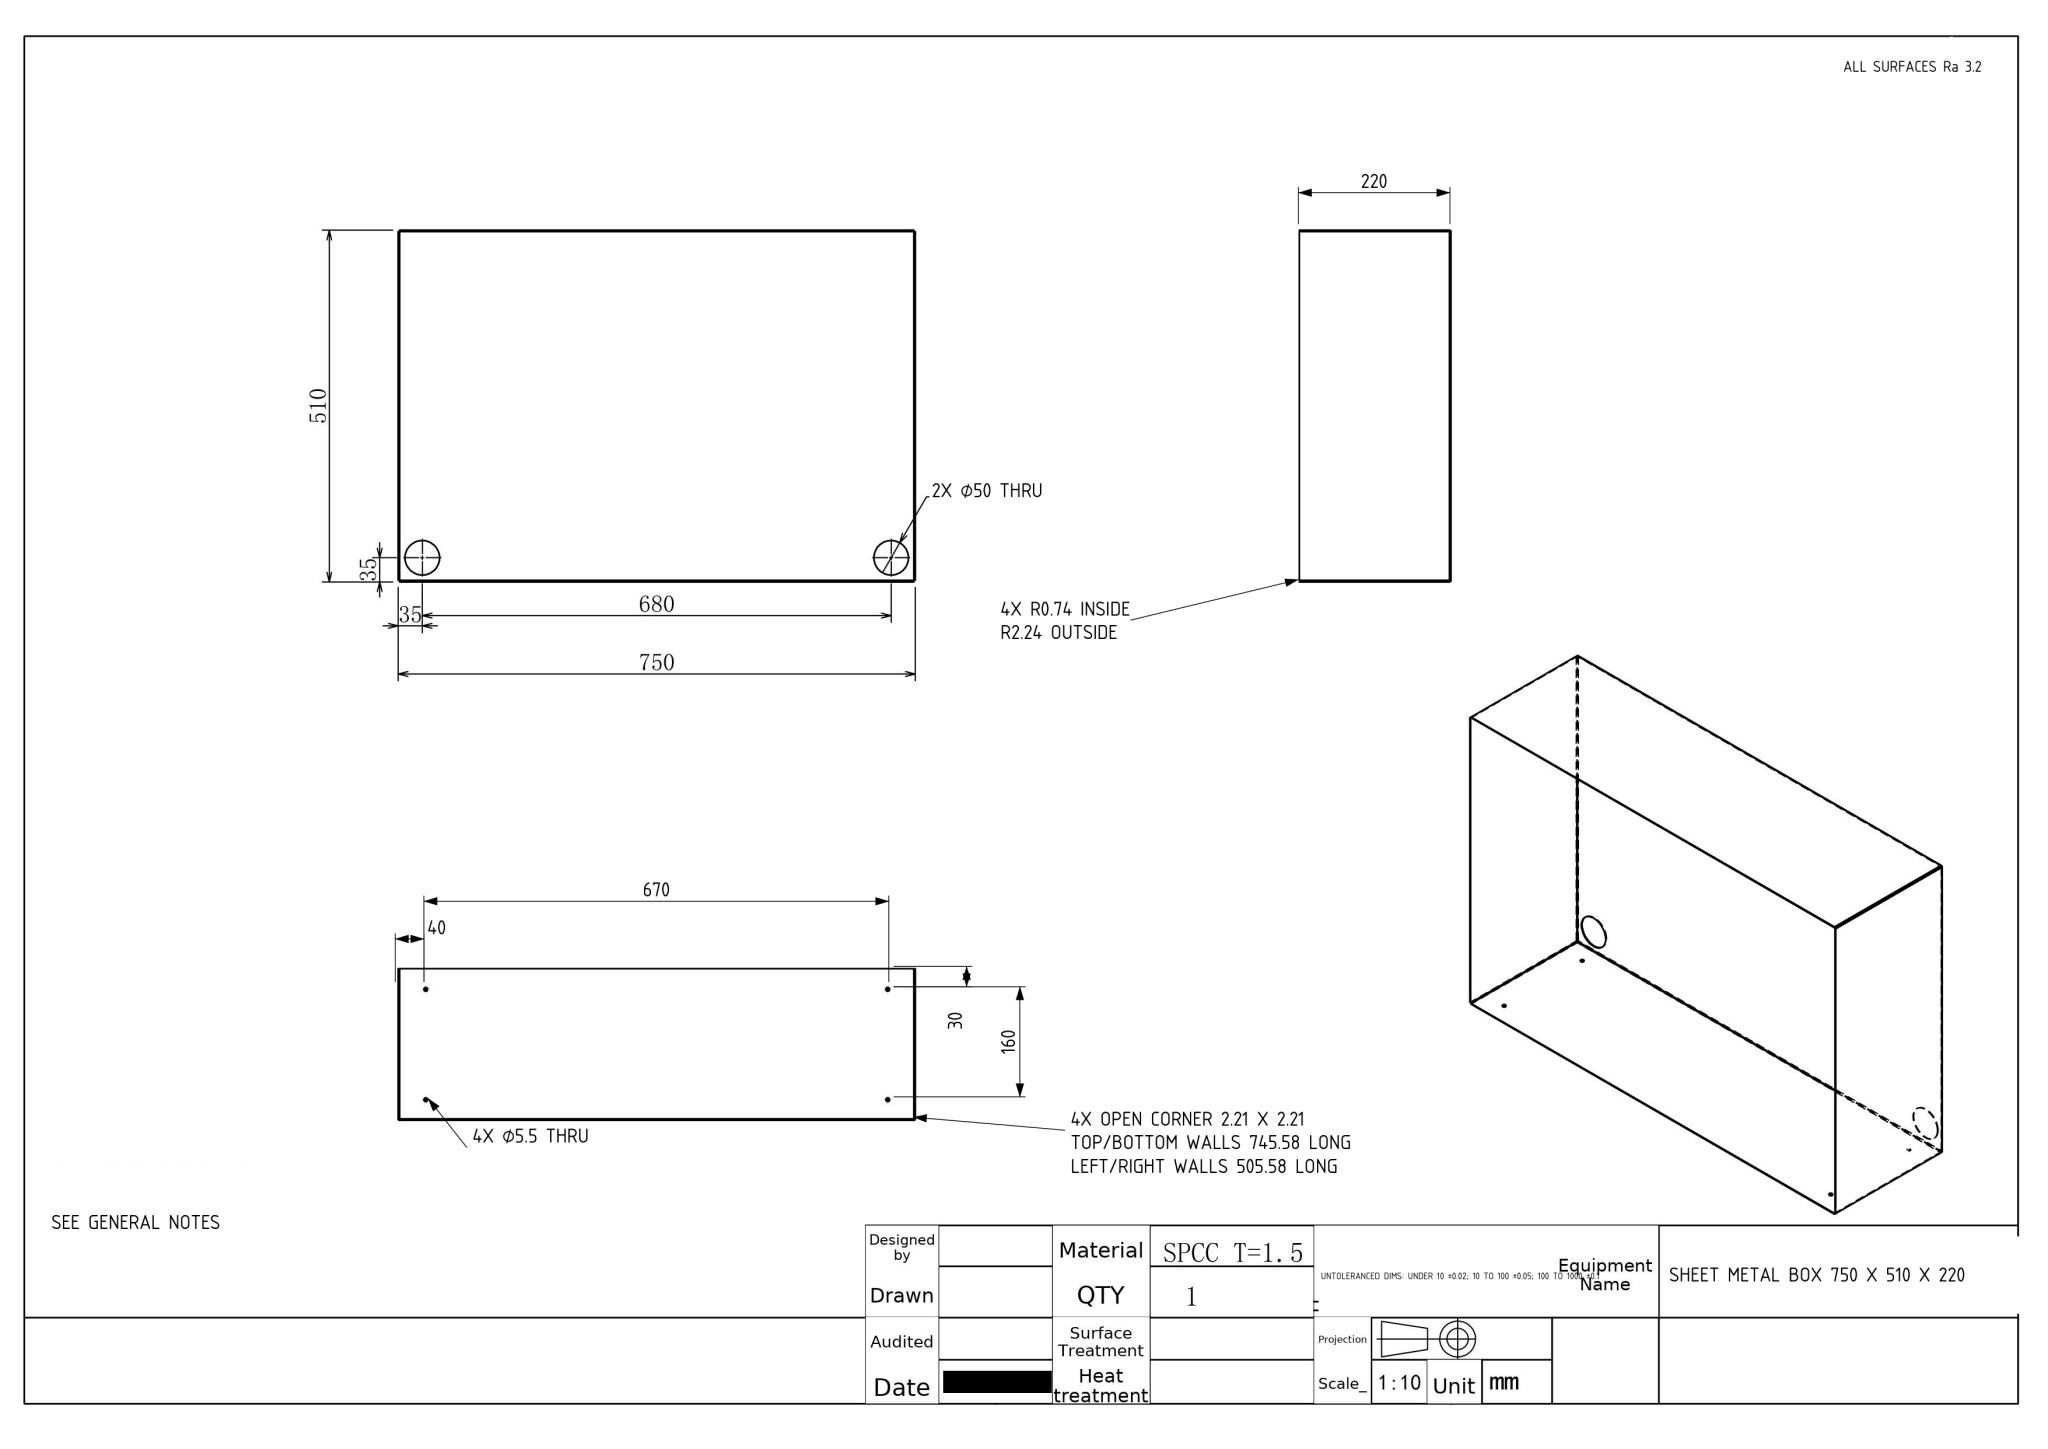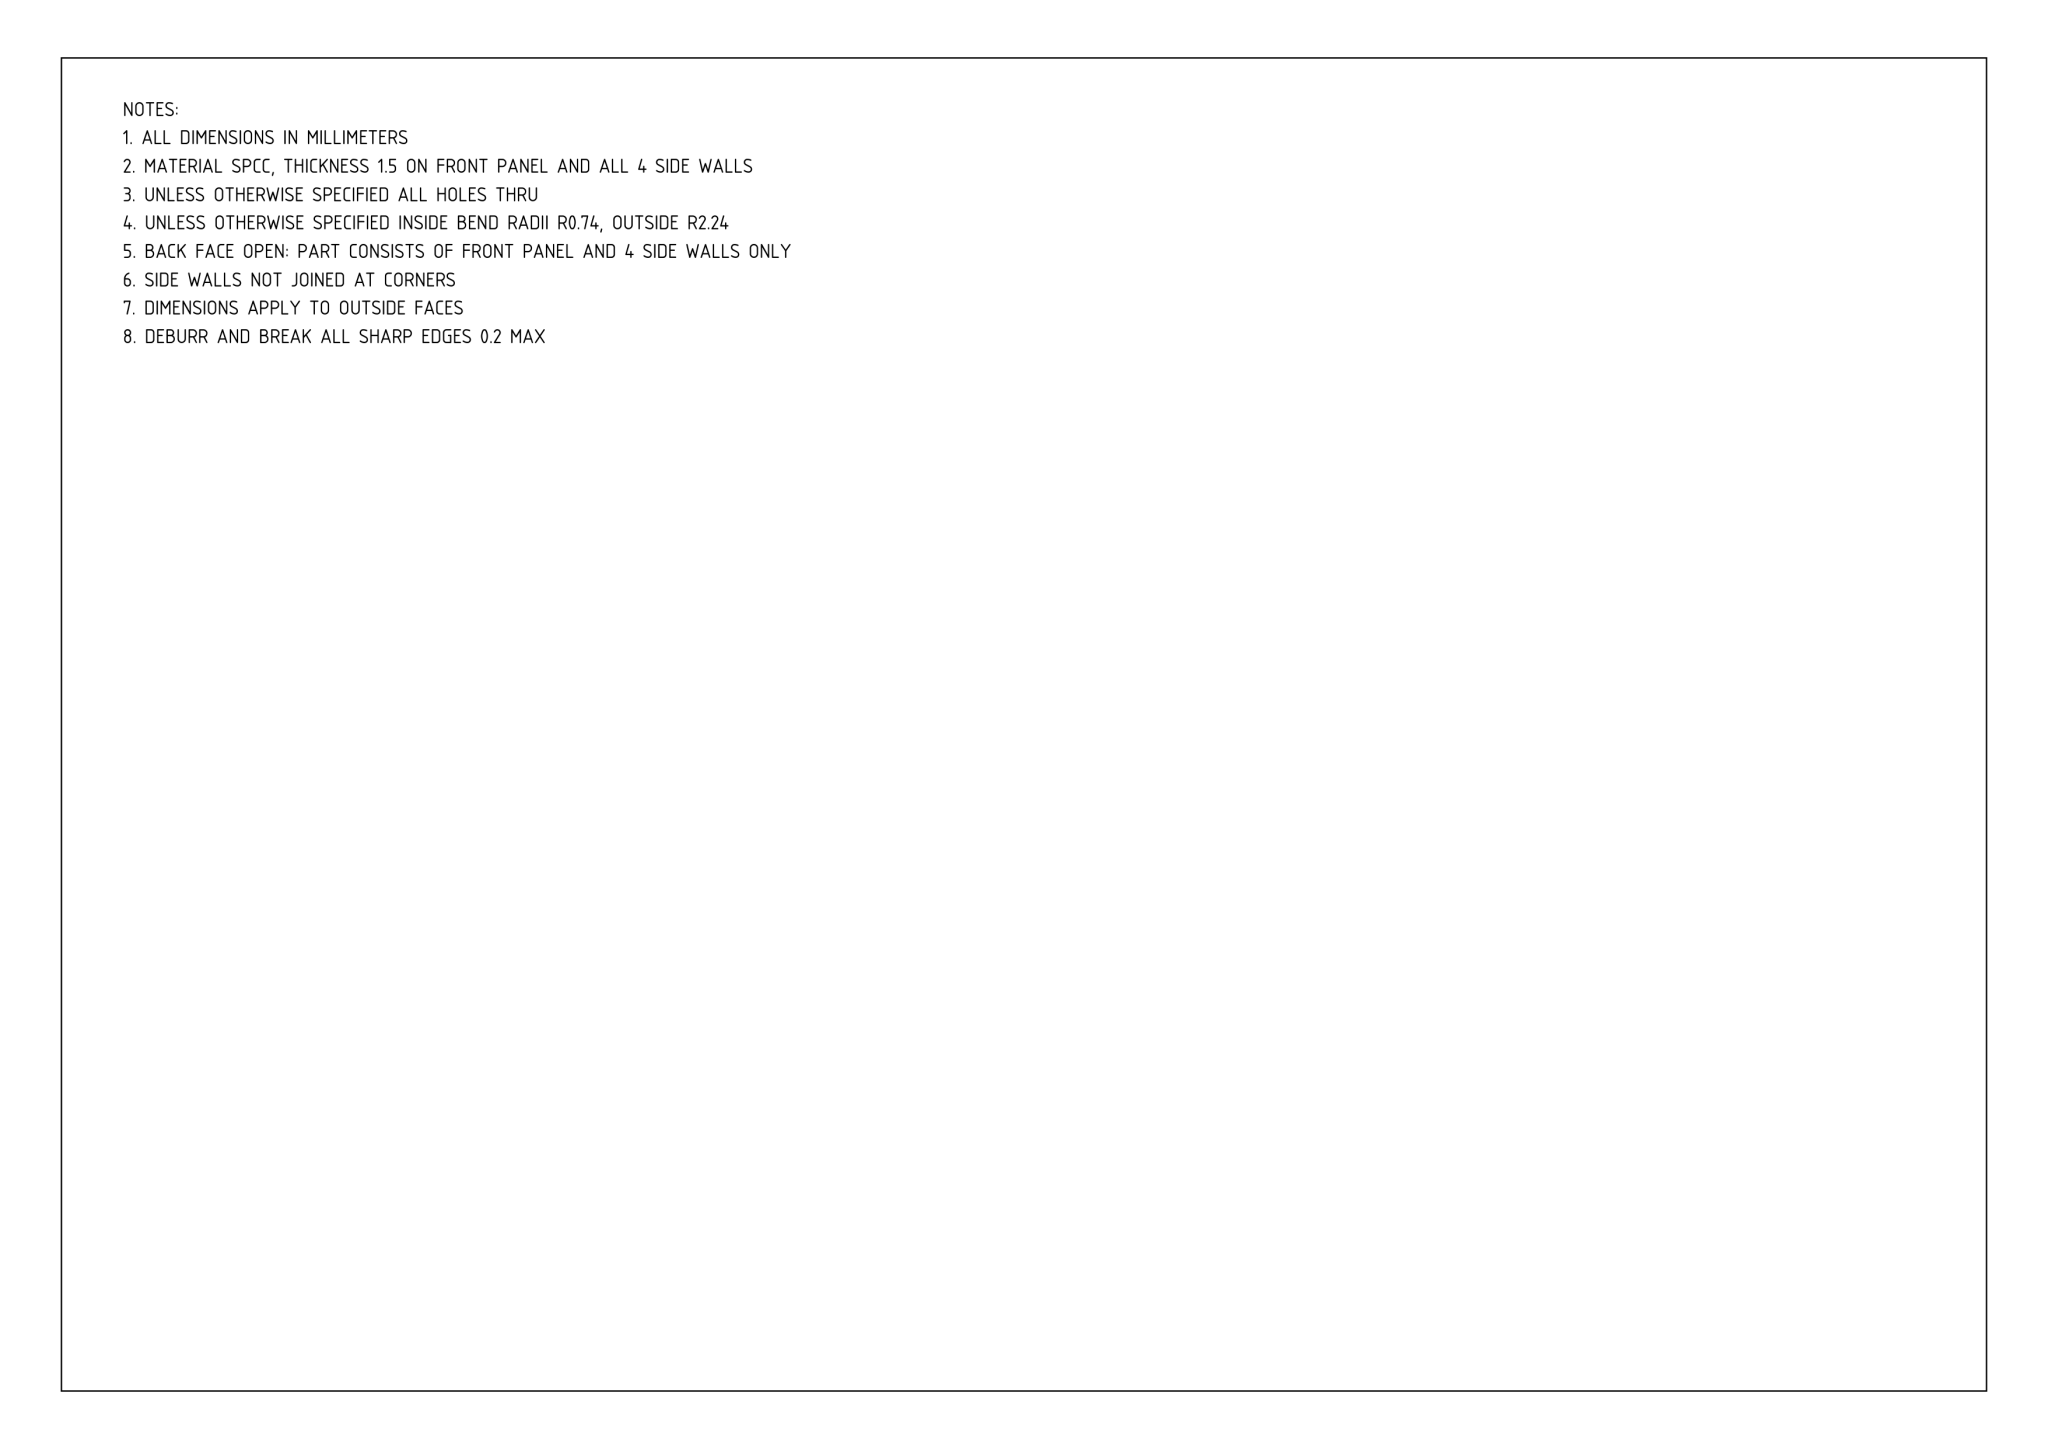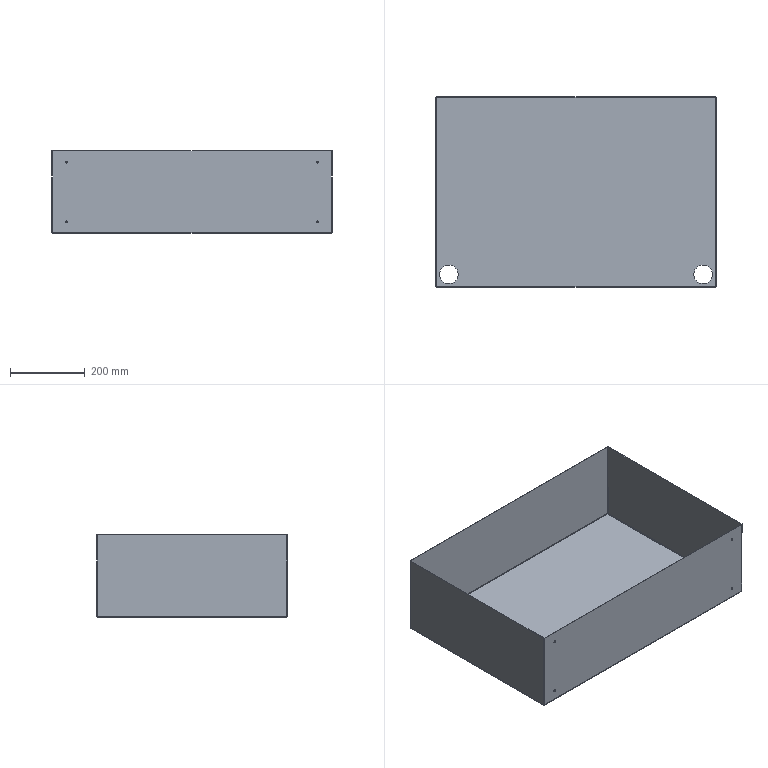Part | NX | mm | 1 solid | 50 faces | box 750 x 510 x 220 mm | volume 1385435 mm3 | plane 22 | cylinder 20 | spline 8 | commonest cylinder face diameters 5.5 x8 50 x4 4.473 x4 1.473 x4